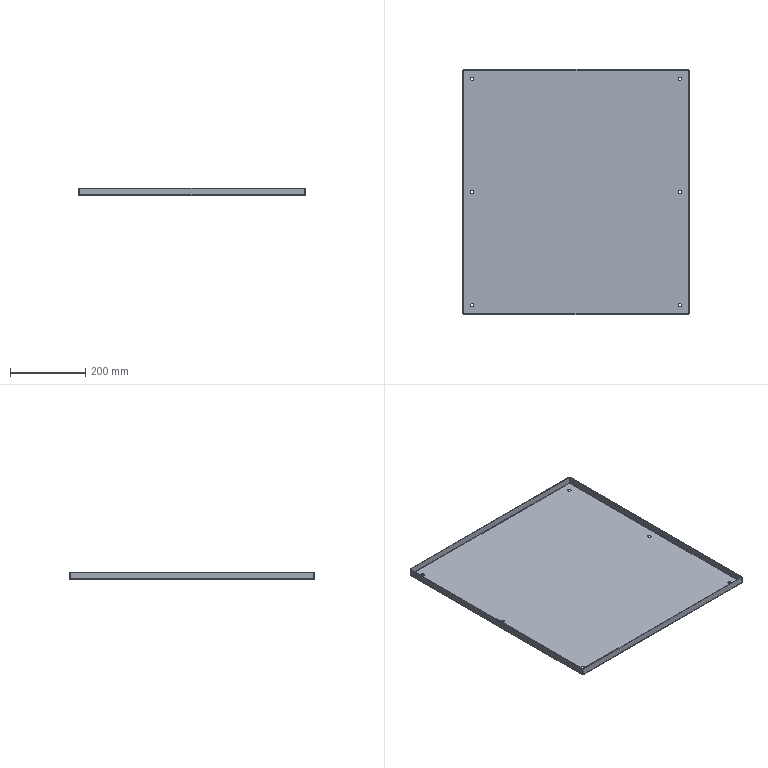Component | SolidWorks | 30-01A-1_ElectricalControlBox-1_ElectricalControlPanel-1 | 1 solid | 50 faces | volume 864703 mm3 | plane 22 | cylinder 20 | spline 8 | commonest cylinder face diameters 9 x12 5.473 x4 1.473 x4